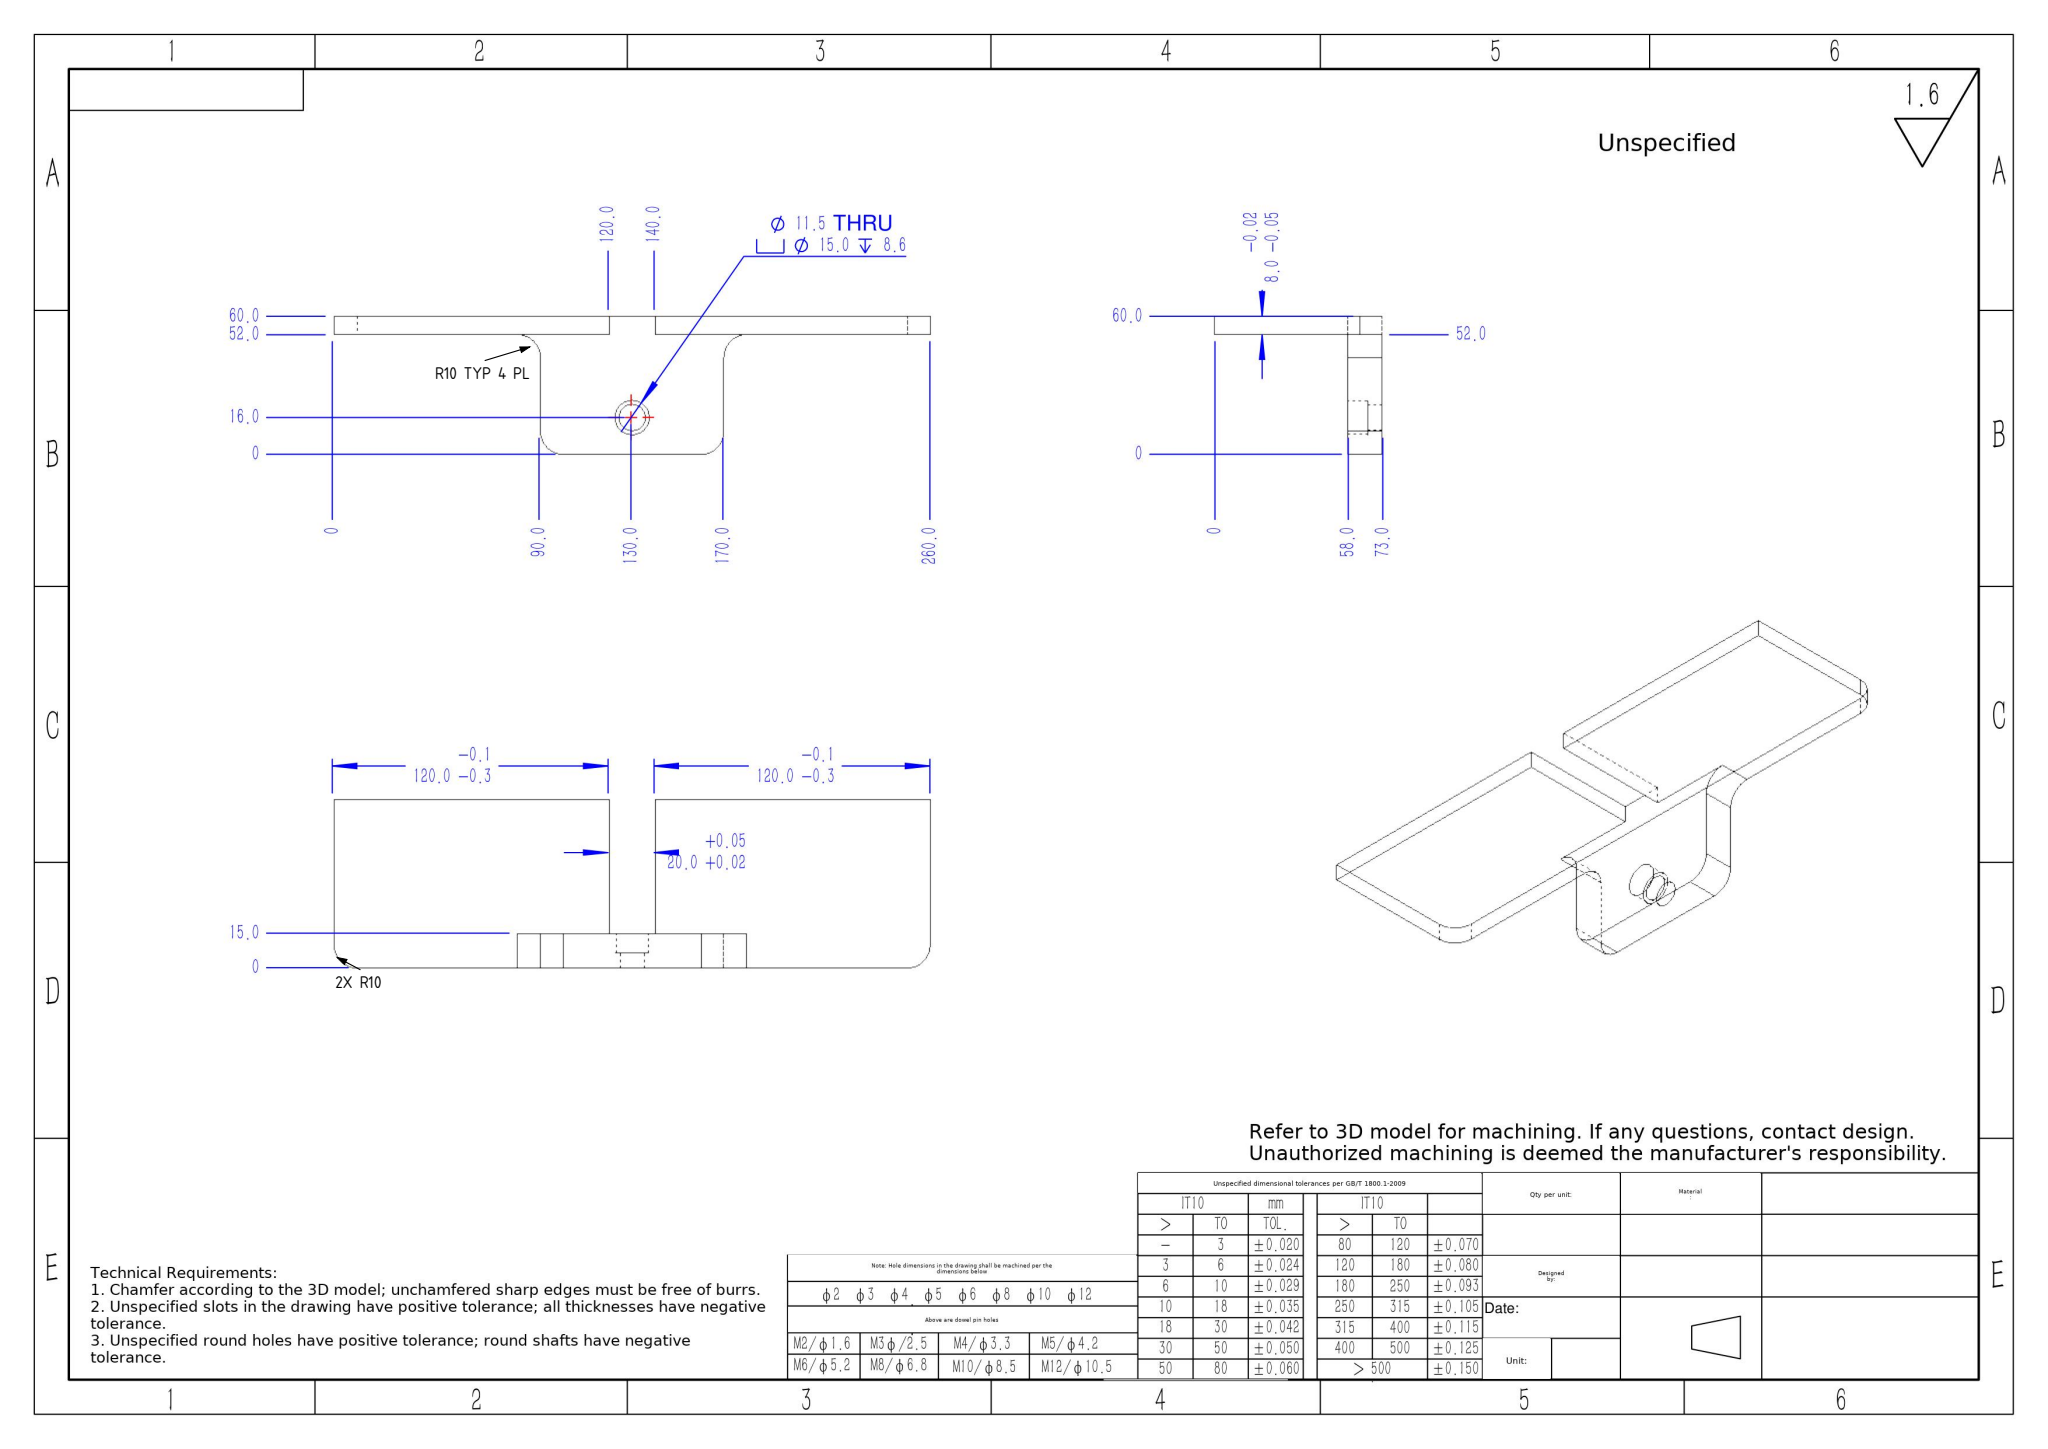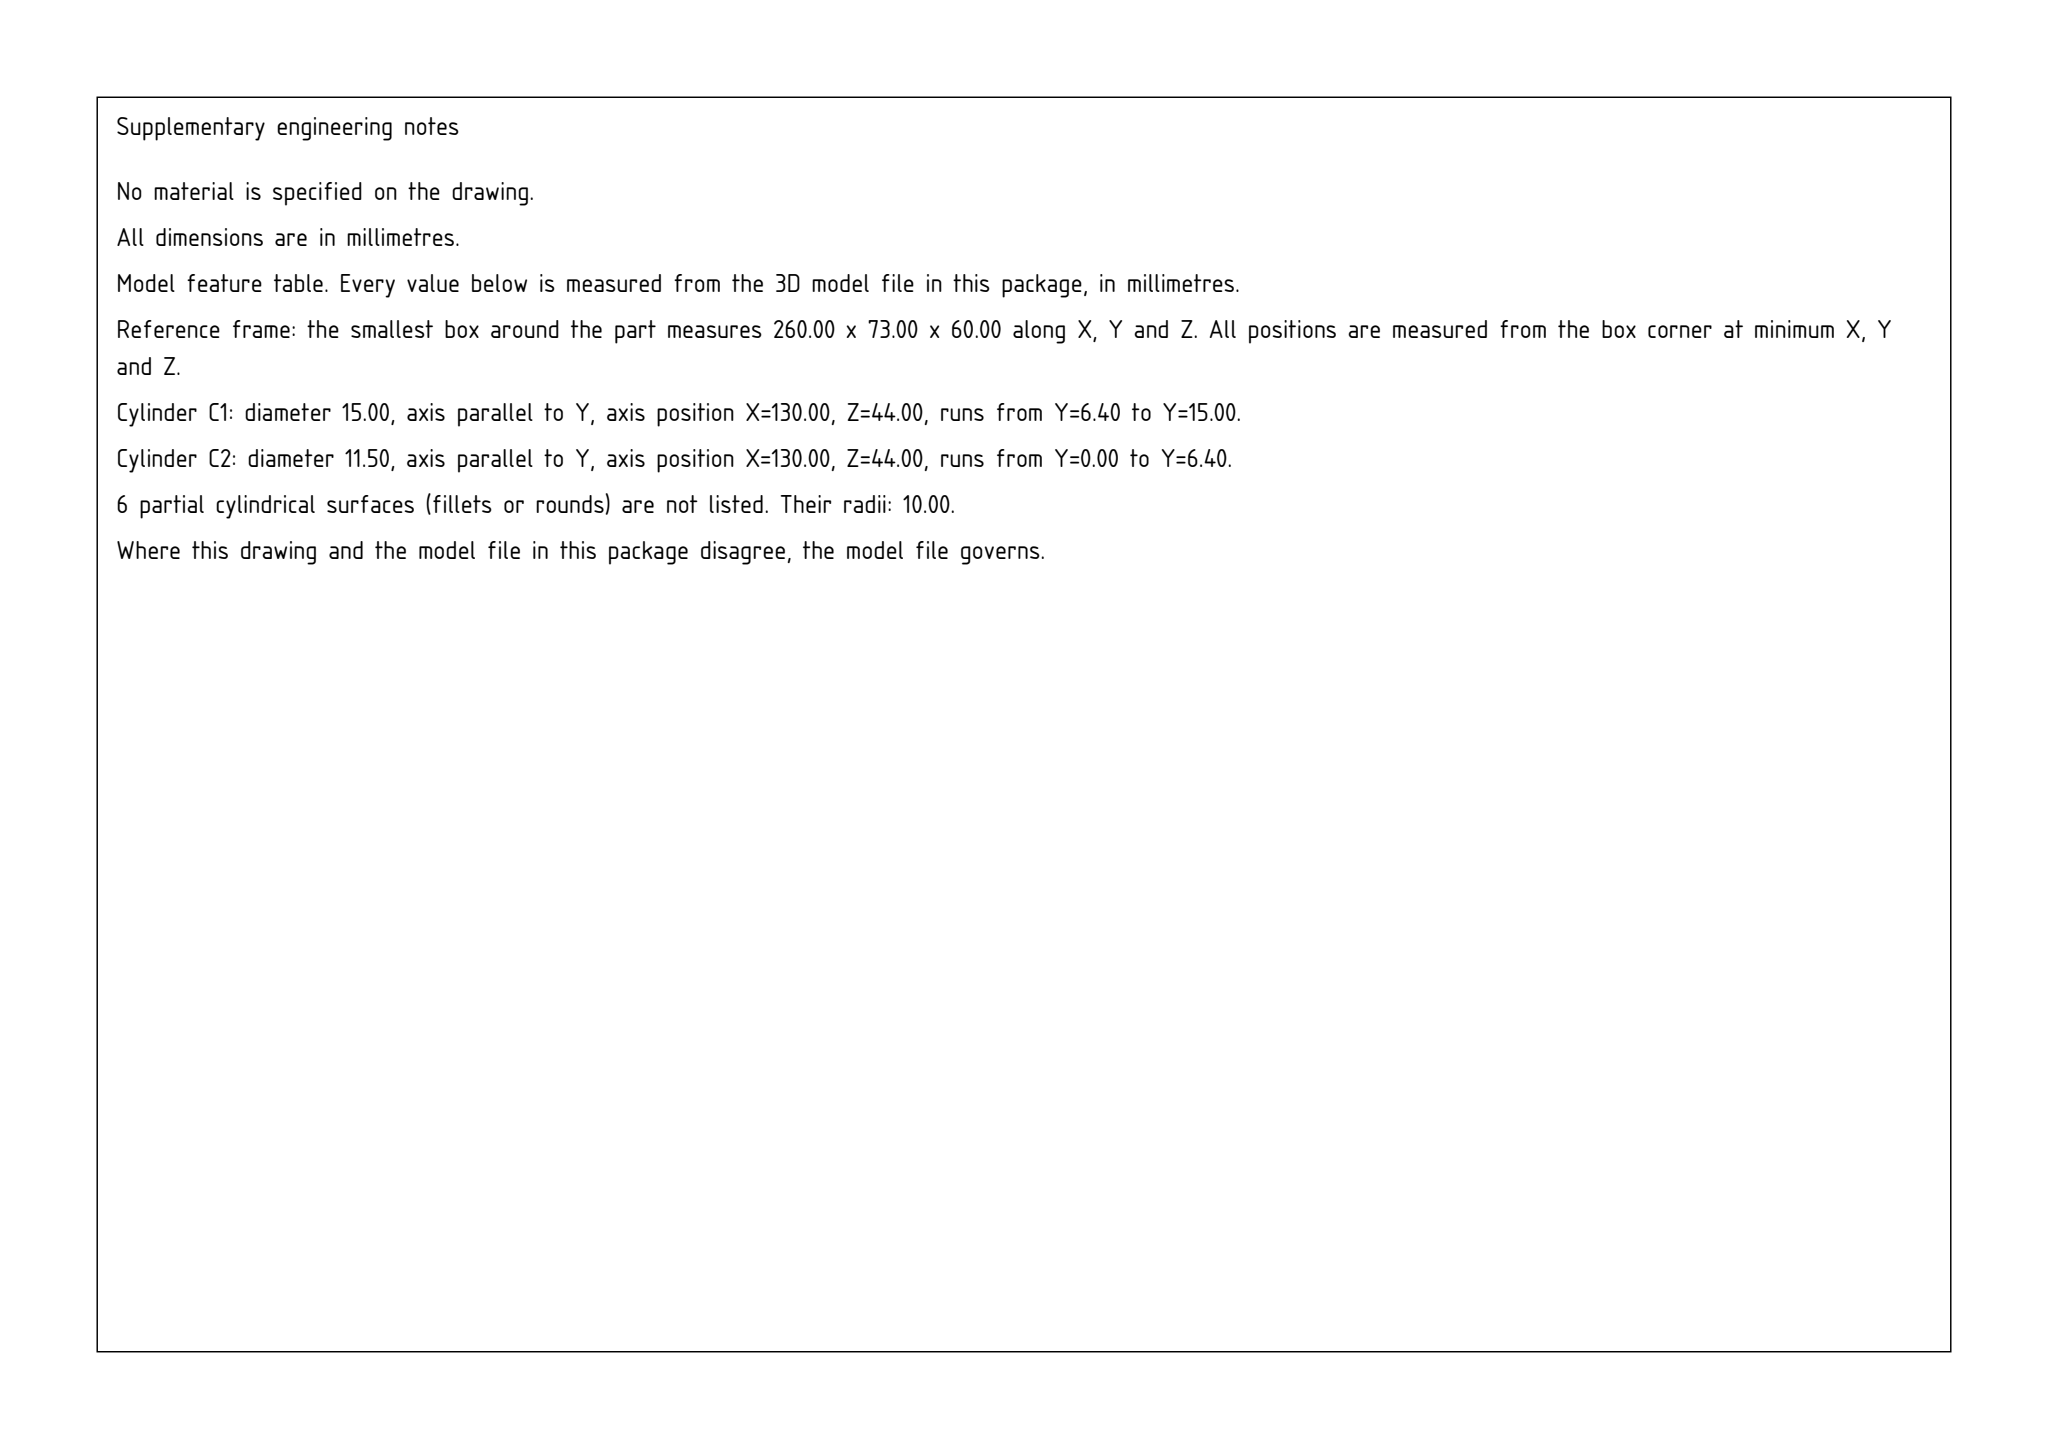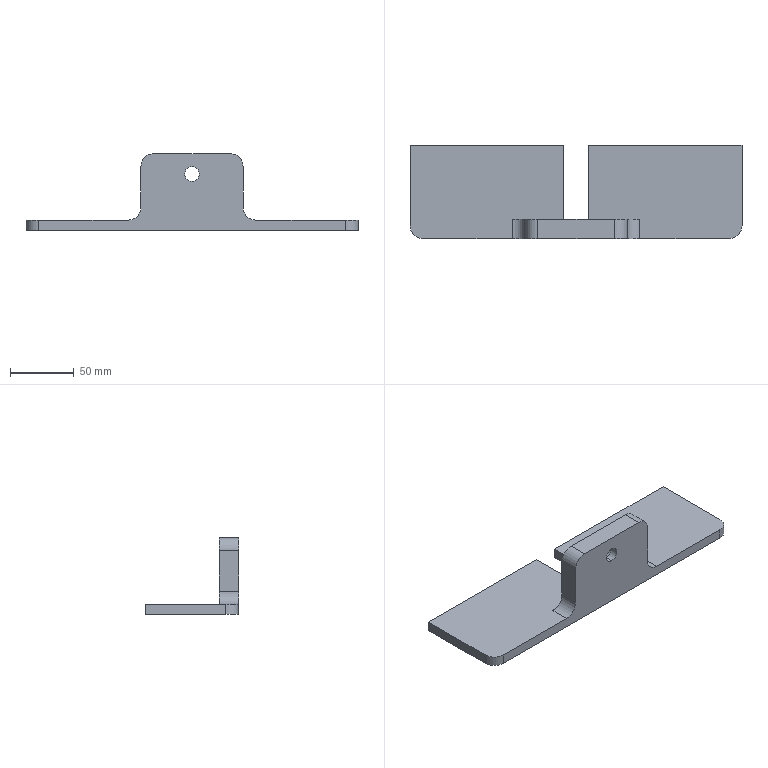Part | SolidWorks | mm | 1 solid | 25 faces | box 260 x 73 x 60 mm | volume 202432 mm3 | plane 15 | cylinder 10 | commonest cylinder face diameters 20 x6 15 x2 11.5 x2
Drawing notes:
R10 TYP 4 PL: WEB-TO-8 THK STRIP BLEND AT X=90 & X=170 | from the solid: cylinders dia 20, axis y, at (x,z)=(80,18),(100,50),(160,50),(180,18), len 15 -> R10 tangent to z=8/z=60 and x=90/170
FRONT VIEW: R10 AT 2 OUTER CORNERS OF 8 THK PLATE (X=0 & 260) | from the solid: cylinders dia 20, axis z, at (x,y)=(10,10),(250,10), len 8 -> R10 tangent to x=0/260 and y=0, thru 8 thk plate
build123d program:
from build123d import *

# Parameters (mm, degrees)
SKETCH1_W                                       = 260
SKETCH1_H                                       = 73
BOSS_EXTRUDE1_DEPTH                             = 30
SKETCH2_W                                       = 52
SKETCH2_H                                       = 58
CUT_EXTRUDE1_DEPTH                              = 265.258
SKETCH3_W                                       = 20
SKETCH3_H                                       = 58
CUT_EXTRUDE2_DEPTH                              = 10
SKETCH4_W                                       = 90
SKETCH4_H                                       = 52
CUT_EXTRUDE3_DEPTH                              = 32
FILLET1_R                                       = 10
FILLET2_R                                       = 10
M8_HEX_SOCKET_HEAD_CAP_SCREW_CBORE1_D           = 11.5
M8_HEX_SOCKET_HEAD_CAP_SCREW_CBORE1_CBORE_D     = 15
M8_HEX_SOCKET_HEAD_CAP_SCREW_CBORE1_CBORE_DEPTH = 8.6


with BuildPart() as part:
    # Sketch1 → Boss-Extrude1 (new, symmetric)
    with BuildSketch(Plane.XY):
        Rectangle(SKETCH1_W, SKETCH1_H)
    extrude(amount=BOSS_EXTRUDE1_DEPTH, both=True)

    # Sketch2 → Cut-Extrude1 (cut, through all)
    with BuildSketch(Plane.ZY.offset(130)):
        with Locations((4, 7.5)):
            Rectangle(SKETCH2_W, SKETCH2_H)
    extrude(amount=-CUT_EXTRUDE1_DEPTH, mode=Mode.SUBTRACT)

    # Sketch3 → Cut-Extrude2 (cut)
    with BuildSketch(Plane.XY.offset(-22)):
        with Locations((0, 7.5)):
            Rectangle(SKETCH3_W, SKETCH3_H)
    extrude(amount=-CUT_EXTRUDE2_DEPTH, mode=Mode.SUBTRACT)

    # Sketch4 → Cut-Extrude3 (cut)
    with BuildSketch(Plane(origin=(0, -21.5, 0), x_dir=(1, 0, 0), z_dir=(0, 1, 0))):
        with Locations((85, -4)):
            Rectangle(SKETCH4_W, SKETCH4_H)
    cut_extrude3 = extrude(amount=-CUT_EXTRUDE3_DEPTH, mode=Mode.SUBTRACT)

    # Mirror1: Cut-Extrude3 across plane
    add(cut_extrude3.mirror(Plane(origin=(0, 0, 0), x_dir=(0, 0, 1), z_dir=(1, 0, 0))), mode=Mode.SUBTRACT)

    # Fillet1
    fillet1_edges = [part.edges().sort_by_distance(p)[0] for p in [
        (40, -29, -22),
        (-40, -29, -22),
    ]]
    fillet(fillet1_edges, radius=FILLET1_R)

    # Fillet2
    fillet2_edges = [part.edges().sort_by_distance(p)[0] for p in [
        (130, -36.5, -26),
        (40, -29, 30),
        (-130, -36.5, -26),
        (-40, -29, 30),
    ]]
    fillet(fillet2_edges, radius=FILLET2_R)

    # M8 Hex Socket Head Cap Screw CBORE1 (through all)
    with Locations(Plane(origin=(0, -21.5, 0), x_dir=(1, 0, 0), z_dir=(0, 1, 0))):
        with Locations((0, -14)):
            CounterBoreHole(M8_HEX_SOCKET_HEAD_CAP_SCREW_CBORE1_D / 2, M8_HEX_SOCKET_HEAD_CAP_SCREW_CBORE1_CBORE_D / 2, M8_HEX_SOCKET_HEAD_CAP_SCREW_CBORE1_CBORE_DEPTH)


solid = part.part
STEP:
#1=CARTESIAN_POINT('',(0.,-30.1,6.5));
#2=VERTEX_POINT('',#1);
#3=CARTESIAN_POINT('',(0.,-30.1,21.5));
#4=VERTEX_POINT('',#3);
#5=CARTESIAN_POINT('',(0.,-30.1,14.));
#6=DIRECTION('',(0.,1.,-0.));
#7=DIRECTION('',(0.,0.,1.));
#8=AXIS2_PLACEMENT_3D('',#5,#6,#7);
#9=CIRCLE('',#8,7.5);
#10=EDGE_CURVE('',#2,#4,#9,.T.);
#11=ORIENTED_EDGE('',*,*,#10,.F.);
#12=CARTESIAN_POINT('',(0.,-21.5,6.5));
#13=VERTEX_POINT('',#12);
#14=CARTESIAN_POINT('',(0.,-21.5,6.5));
#15=DIRECTION('',(0.,1.,-0.));
#16=VECTOR('',#15,1000.);
#17=LINE('',#14,#16);
#18=EDGE_CURVE('',#2,#13,#17,.T.);
#19=ORIENTED_EDGE('',*,*,#18,.T.);
#20=CARTESIAN_POINT('',(0.,-21.5,21.5));
#21=VERTEX_POINT('',#20);
#22=CARTESIAN_POINT('',(0.,-21.5,14.));
#23=DIRECTION('',(0.,1.,-0.));
#24=DIRECTION('',(0.,0.,1.));
#25=AXIS2_PLACEMENT_3D('',#22,#23,#24);
#26=CIRCLE('',#25,7.5);
#27=EDGE_CURVE('',#13,#21,#26,.T.);
#28=ORIENTED_EDGE('',*,*,#27,.T.);
#29=CARTESIAN_POINT('',(0.,-21.5,21.5));
#30=DIRECTION('',(0.,1.,-0.));
#31=VECTOR('',#30,1000.);
#32=LINE('',#29,#31);
#33=EDGE_CURVE('',#4,#21,#32,.T.);
#34=ORIENTED_EDGE('',*,*,#33,.F.);
#35=EDGE_LOOP('',(#11,#19,#28,#34));
#36=FACE_OUTER_BOUND('',#35,.T.);
#37=CARTESIAN_POINT('',(0.,-21.5,14.));
#38=DIRECTION('',(0.,1.,-0.));
#39=DIRECTION('',(0.,0.,1.));
#40=AXIS2_PLACEMENT_3D('',#37,#38,#39);
#41=CYLINDRICAL_SURFACE('',#40,7.5);
#42=ADVANCED_FACE('',(#36),#41,.F.);
#43=CARTESIAN_POINT('',(0.,-36.5,8.25));
#44=VERTEX_POINT('',#43);
#45=CARTESIAN_POINT('',(0.,-36.5,19.75));
#46=VERTEX_POINT('',#45);
#47=CARTESIAN_POINT('',(0.,-36.5,14.));
#48=DIRECTION('',(0.,1.,-0.));
#49=DIRECTION('',(0.,0.,1.));
#50=AXIS2_PLACEMENT_3D('',#47,#48,#49);
#51=CIRCLE('',#50,5.75);
#52=EDGE_CURVE('',#44,#46,#51,.T.);
#53=ORIENTED_EDGE('',*,*,#52,.F.);
#54=CARTESIAN_POINT('',(0.,-30.1,8.25));
#55=VERTEX_POINT('',#54);
#56=CARTESIAN_POINT('',(0.,-21.5,8.25));
#57=DIRECTION('',(0.,1.,-0.));
#58=VECTOR('',#57,1000.);
#59=LINE('',#56,#58);
#60=EDGE_CURVE('',#44,#55,#59,.T.);
#61=ORIENTED_EDGE('',*,*,#60,.T.);
#62=CARTESIAN_POINT('',(0.,-30.1,19.75));
#63=VERTEX_POINT('',#62);
#64=CARTESIAN_POINT('',(0.,-30.1,14.));
#65=DIRECTION('',(0.,1.,-0.));
#66=DIRECTION('',(0.,0.,1.));
#67=AXIS2_PLACEMENT_3D('',#64,#65,#66);
#68=CIRCLE('',#67,5.75);
#69=EDGE_CURVE('',#55,#63,#68,.T.);
#70=ORIENTED_EDGE('',*,*,#69,.T.);
#71=CARTESIAN_POINT('',(0.,-21.5,19.75));
#72=DIRECTION('',(0.,1.,-0.));
#73=VECTOR('',#72,1000.);
#74=LINE('',#71,#73);
#75=EDGE_CURVE('',#46,#63,#74,.T.);
#76=ORIENTED_EDGE('',*,*,#75,.F.);
#77=EDGE_LOOP('',(#53,#61,#70,#76));
#78=FACE_OUTER_BOUND('',#77,.T.);
#79=CARTESIAN_POINT('',(0.,-21.5,14.));
#80=DIRECTION('',(0.,1.,-0.));
#81=DIRECTION('',(0.,0.,1.));
#82=AXIS2_PLACEMENT_3D('',#79,#80,#81);
#83=CYLINDRICAL_SURFACE('',#82,5.75);
#84=ADVANCED_FACE('',(#78),#83,.F.);
#85=CARTESIAN_POINT('',(-130.,36.5,-30.));
#86=VERTEX_POINT('',#85);
#87=CARTESIAN_POINT('',(-130.,-26.5,-30.));
#88=VERTEX_POINT('',#87);
#89=CARTESIAN_POINT('',(-130.,-36.5,-30.));
#90=DIRECTION('',(0.,-1.,0.));
#91=VECTOR('',#90,1000.);
#92=LINE('',#89,#91);
#93=EDGE_CURVE('',#86,#88,#92,.T.);
#94=ORIENTED_EDGE('',*,*,#93,.T.);
#95=CARTESIAN_POINT('',(-130.,-26.5,-22.));
#96=VERTEX_POINT('',#95);
#97=CARTESIAN_POINT('',(-130.,-26.5,30.));
#98=DIRECTION('',(0.,0.,1.));
#99=VECTOR('',#98,1000.);
#100=LINE('',#97,#99);
#101=EDGE_CURVE('',#88,#96,#100,.T.);
#102=ORIENTED_EDGE('',*,*,#101,.T.);
#103=CARTESIAN_POINT('',(-130.,36.5,-22.));
#104=VERTEX_POINT('',#103);
#105=CARTESIAN_POINT('',(-130.,36.5,-22.));
#106=DIRECTION('',(0.,-1.,0.));
#107=VECTOR('',#106,1000.);
#108=LINE('',#105,#107);
#109=EDGE_CURVE('',#104,#96,#108,.T.);
#110=ORIENTED_EDGE('',*,*,#109,.F.);
#111=CARTESIAN_POINT('',(-130.,36.5,30.));
#112=DIRECTION('',(0.,0.,-1.));
#113=VECTOR('',#112,1000.);
#114=LINE('',#111,#113);
#115=EDGE_CURVE('',#104,#86,#114,.T.);
#116=ORIENTED_EDGE('',*,*,#115,.T.);
#117=EDGE_LOOP('',(#94,#102,#110,#116));
#118=FACE_OUTER_BOUND('',#117,.T.);
#119=CARTESIAN_POINT('',(-130.,-36.5,30.));
#120=DIRECTION('',(1.,0.,0.));
#121=DIRECTION('',(0.,0.,-1.));
#122=AXIS2_PLACEMENT_3D('',#119,#120,#121);
#123=PLANE('',#122);
#124=ADVANCED_FACE('',(#118),#123,.F.);
#125=CARTESIAN_POINT('',(0.,-36.5,14.));
#126=DIRECTION('',(0.,1.,-0.));
#127=DIRECTION('',(0.,0.,1.));
#128=AXIS2_PLACEMENT_3D('',#125,#126,#127);
#129=CIRCLE('',#128,5.75);
#130=EDGE_CURVE('',#46,#44,#129,.T.);
#131=ORIENTED_EDGE('',*,*,#130,.T.);
#132=ORIENTED_EDGE('',*,*,#52,.T.);
#133=EDGE_LOOP('',(#131,#132));
#134=FACE_BOUND('',#133,.T.);
#135=CARTESIAN_POINT('',(-30.,-36.5,30.));
#136=VERTEX_POINT('',#135);
#137=CARTESIAN_POINT('',(30.,-36.5,30.));
#138=VERTEX_POINT('',#137);
#139=CARTESIAN_POINT('',(-130.,-36.5,30.));
#140=DIRECTION('',(1.,0.,0.));
#141=VECTOR('',#140,1000.);
#142=LINE('',#139,#141);
#143=EDGE_CURVE('',#136,#138,#142,.T.);
#144=ORIENTED_EDGE('',*,*,#143,.F.);
#145=CARTESIAN_POINT('',(-40.,-36.5,20.));
#146=VERTEX_POINT('',#145);
#147=CARTESIAN_POINT('',(-30.,-36.5,20.));
#148=DIRECTION('',(0.,-1.,0.));
#149=DIRECTION('',(0.,0.,1.));
#150=AXIS2_PLACEMENT_3D('',#147,#148,#149);
#151=CIRCLE('',#150,10.);
#152=EDGE_CURVE('',#136,#146,#151,.T.);
#153=ORIENTED_EDGE('',*,*,#152,.T.);
#154=CARTESIAN_POINT('',(-40.,-36.5,-12.));
#155=VERTEX_POINT('',#154);
#156=CARTESIAN_POINT('',(-40.,-36.5,30.));
#157=DIRECTION('',(0.,0.,1.));
#158=VECTOR('',#157,1000.);
#159=LINE('',#156,#158);
#160=EDGE_CURVE('',#155,#146,#159,.T.);
#161=ORIENTED_EDGE('',*,*,#160,.F.);
#162=CARTESIAN_POINT('',(-50.,-36.5,-22.));
#163=VERTEX_POINT('',#162);
#164=CARTESIAN_POINT('',(-50.,-36.5,-12.));
#165=DIRECTION('',(0.,1.,0.));
#166=DIRECTION('',(0.,0.,1.));
#167=AXIS2_PLACEMENT_3D('',#164,#165,#166);
#168=CIRCLE('',#167,10.);
#169=EDGE_CURVE('',#155,#163,#168,.T.);
#170=ORIENTED_EDGE('',*,*,#169,.T.);
#171=CARTESIAN_POINT('',(-120.,-36.5,-22.));
#172=VERTEX_POINT('',#171);
#173=CARTESIAN_POINT('',(-130.,-36.5,-22.));
#174=DIRECTION('',(1.,0.,0.));
#175=VECTOR('',#174,1000.);
#176=LINE('',#173,#175);
#177=EDGE_CURVE('',#172,#163,#176,.T.);
#178=ORIENTED_EDGE('',*,*,#177,.F.);
#179=CARTESIAN_POINT('',(-120.,-36.5,-30.));
#180=VERTEX_POINT('',#179);
#181=CARTESIAN_POINT('',(-120.,-36.5,30.));
#182=DIRECTION('',(0.,0.,-1.));
#183=VECTOR('',#182,1000.);
#184=LINE('',#181,#183);
#185=EDGE_CURVE('',#172,#180,#184,.T.);
#186=ORIENTED_EDGE('',*,*,#185,.T.);
#187=CARTESIAN_POINT('',(120.,-36.5,-30.));
#188=VERTEX_POINT('',#187);
#189=CARTESIAN_POINT('',(-130.,-36.5,-30.));
#190=DIRECTION('',(1.,0.,0.));
#191=VECTOR('',#190,1000.);
#192=LINE('',#189,#191);
#193=EDGE_CURVE('',#180,#188,#192,.T.);
#194=ORIENTED_EDGE('',*,*,#193,.T.);
#195=CARTESIAN_POINT('',(120.,-36.5,-22.));
#196=VERTEX_POINT('',#195);
#197=CARTESIAN_POINT('',(120.,-36.5,30.));
#198=DIRECTION('',(0.,0.,1.));
#199=VECTOR('',#198,1000.);
#200=LINE('',#197,#199);
#201=EDGE_CURVE('',#188,#196,#200,.T.);
#202=ORIENTED_EDGE('',*,*,#201,.T.);
#203=CARTESIAN_POINT('',(50.,-36.5,-22.));
#204=VERTEX_POINT('',#203);
#205=CARTESIAN_POINT('',(-130.,-36.5,-22.));
#206=DIRECTION('',(-1.,0.,0.));
#207=VECTOR('',#206,1000.);
#208=LINE('',#205,#207);
#209=EDGE_CURVE('',#196,#204,#208,.T.);
#210=ORIENTED_EDGE('',*,*,#209,.T.);
#211=CARTESIAN_POINT('',(40.,-36.5,-12.));
#212=VERTEX_POINT('',#211);
#213=CARTESIAN_POINT('',(50.,-36.5,-12.));
#214=DIRECTION('',(0.,1.,0.));
#215=DIRECTION('',(0.,0.,1.));
#216=AXIS2_PLACEMENT_3D('',#213,#214,#215);
#217=CIRCLE('',#216,10.);
#218=EDGE_CURVE('',#204,#212,#217,.T.);
#219=ORIENTED_EDGE('',*,*,#218,.T.);
#220=CARTESIAN_POINT('',(40.,-36.5,20.));
#221=VERTEX_POINT('',#220);
#222=CARTESIAN_POINT('',(40.,-36.5,30.));
#223=DIRECTION('',(0.,0.,1.));
#224=VECTOR('',#223,1000.);
#225=LINE('',#222,#224);
#226=EDGE_CURVE('',#212,#221,#225,.T.);
#227=ORIENTED_EDGE('',*,*,#226,.T.);
#228=CARTESIAN_POINT('',(30.,-36.5,20.));
#229=DIRECTION('',(0.,-1.,0.));
#230=DIRECTION('',(0.,0.,1.));
#231=AXIS2_PLACEMENT_3D('',#228,#229,#230);
#232=CIRCLE('',#231,10.);
#233=EDGE_CURVE('',#221,#138,#232,.T.);
#234=ORIENTED_EDGE('',*,*,#233,.T.);
#235=EDGE_LOOP('',(#144,#153,#161,#170,#178,#186,#194,#202,#210,#219,#227,#234));
#236=FACE_OUTER_BOUND('',#235,.T.);
#237=CARTESIAN_POINT('',(-130.,-36.5,30.));
#238=DIRECTION('',(0.,1.,0.));
#239=DIRECTION('',(0.,0.,1.));
#240=AXIS2_PLACEMENT_3D('',#237,#238,#239);
#241=PLANE('',#240);
#242=ADVANCED_FACE('',(#134,#236),#241,.F.);
#243=CARTESIAN_POINT('',(30.,-21.5,30.));
#244=VERTEX_POINT('',#243);
#245=CARTESIAN_POINT('',(-30.,-21.5,30.));
#246=VERTEX_POINT('',#245);
#247=CARTESIAN_POINT('',(130.,-21.5,30.));
#248=DIRECTION('',(-1.,0.,0.));
#249=VECTOR('',#248,1000.);
#250=LINE('',#247,#249);
#251=EDGE_CURVE('',#244,#246,#250,.T.);
#252=ORIENTED_EDGE('',*,*,#251,.T.);
#253=CARTESIAN_POINT('',(-30.,-36.5,30.));
#254=DIRECTION('',(0.,-1.,0.));
#255=VECTOR('',#254,1000.);
#256=LINE('',#253,#255);
#257=EDGE_CURVE('',#246,#136,#256,.T.);
#258=ORIENTED_EDGE('',*,*,#257,.T.);
#259=ORIENTED_EDGE('',*,*,#143,.T.);
#260=CARTESIAN_POINT('',(30.,0.,30.));
#261=DIRECTION('',(0.,1.,0.));
#262=VECTOR('',#261,1000.);
#263=LINE('',#260,#262);
#264=EDGE_CURVE('',#138,#244,#263,.T.);
#265=ORIENTED_EDGE('',*,*,#264,.T.);
#266=EDGE_LOOP('',(#252,#258,#259,#265));
#267=FACE_OUTER_BOUND('',#266,.T.);
#268=CARTESIAN_POINT('',(0.,0.,30.));
#269=DIRECTION('',(0.,0.,-1.));
#270=DIRECTION('',(-1.,0.,0.));
#271=AXIS2_PLACEMENT_3D('',#268,#269,#270);
#272=PLANE('',#271);
#273=ADVANCED_FACE('',(#267),#272,.F.);
#274=CARTESIAN_POINT('',(0.,-21.5,14.));
#275=DIRECTION('',(0.,1.,-0.));
#276=DIRECTION('',(0.,0.,1.));
#277=AXIS2_PLACEMENT_3D('',#274,#275,#276);
#278=CIRCLE('',#277,7.5);
#279=EDGE_CURVE('',#21,#13,#278,.T.);
#280=ORIENTED_EDGE('',*,*,#279,.F.);
#281=ORIENTED_EDGE('',*,*,#27,.F.);
#282=EDGE_LOOP('',(#280,#281));
#283=FACE_BOUND('',#282,.T.);
#284=CARTESIAN_POINT('',(-40.,-21.5,-12.));
#285=VERTEX_POINT('',#284);
#286=CARTESIAN_POINT('',(-40.,-21.5,20.));
#287=VERTEX_POINT('',#286);
#288=CARTESIAN_POINT('',(-40.,-21.5,30.));
#289=DIRECTION('',(0.,0.,1.));
#290=VECTOR('',#289,1000.);
#291=LINE('',#288,#290);
#292=EDGE_CURVE('',#285,#287,#291,.T.);
#293=ORIENTED_EDGE('',*,*,#292,.T.);
#294=CARTESIAN_POINT('',(-30.,-21.5,20.));
#295=DIRECTION('',(0.,1.,-0.));
#296=DIRECTION('',(0.,0.,-1.));
#297=AXIS2_PLACEMENT_3D('',#294,#295,#296);
#298=CIRCLE('',#297,10.);
#299=EDGE_CURVE('',#287,#246,#298,.T.);
#300=ORIENTED_EDGE('',*,*,#299,.T.);
#301=ORIENTED_EDGE('',*,*,#251,.F.);
#302=CARTESIAN_POINT('',(40.,-21.5,20.));
#303=VERTEX_POINT('',#302);
#304=CARTESIAN_POINT('',(30.,-21.5,20.));
#305=DIRECTION('',(0.,1.,-0.));
#306=DIRECTION('',(0.,0.,-1.));
#307=AXIS2_PLACEMENT_3D('',#304,#305,#306);
#308=CIRCLE('',#307,10.);
#309=EDGE_CURVE('',#244,#303,#308,.T.);
#310=ORIENTED_EDGE('',*,*,#309,.T.);
#311=CARTESIAN_POINT('',(40.,-21.5,-12.));
#312=VERTEX_POINT('',#311);
#313=CARTESIAN_POINT('',(40.,-21.5,30.));
#314=DIRECTION('',(0.,0.,1.));
#315=VECTOR('',#314,1000.);
#316=LINE('',#313,#315);
#317=EDGE_CURVE('',#312,#303,#316,.T.);
#318=ORIENTED_EDGE('',*,*,#317,.F.);
#319=CARTESIAN_POINT('',(50.,-21.5,-22.));
#320=VERTEX_POINT('',#319);
#321=CARTESIAN_POINT('',(50.,-21.5,-12.));
#322=DIRECTION('',(0.,-1.,0.));
#323=DIRECTION('',(0.,0.,-1.));
#324=AXIS2_PLACEMENT_3D('',#321,#322,#323);
#325=CIRCLE('',#324,10.);
#326=EDGE_CURVE('',#312,#320,#325,.T.);
#327=ORIENTED_EDGE('',*,*,#326,.T.);
#328=CARTESIAN_POINT('',(10.,-21.5,-22.));
#329=VERTEX_POINT('',#328);
#330=CARTESIAN_POINT('',(130.,-21.5,-22.));
#331=DIRECTION('',(-1.,0.,0.));
#332=VECTOR('',#331,1000.);
#333=LINE('',#330,#332);
#334=EDGE_CURVE('',#320,#329,#333,.T.);
#335=ORIENTED_EDGE('',*,*,#334,.T.);
#336=CARTESIAN_POINT('',(10.,-21.5,-30.));
#337=VERTEX_POINT('',#336);
#338=CARTESIAN_POINT('',(10.,-21.5,-32.));
#339=DIRECTION('',(0.,0.,1.));
#340=VECTOR('',#339,1000.);
#341=LINE('',#338,#340);
#342=EDGE_CURVE('',#337,#329,#341,.T.);
#343=ORIENTED_EDGE('',*,*,#342,.F.);
#344=CARTESIAN_POINT('',(-10.,-21.5,-30.));
#345=VERTEX_POINT('',#344);
#346=CARTESIAN_POINT('',(0.,-21.5,-30.));
#347=DIRECTION('',(-1.,0.,0.));
#348=VECTOR('',#347,1000.);
#349=LINE('',#346,#348);
#350=EDGE_CURVE('',#337,#345,#349,.T.);
#351=ORIENTED_EDGE('',*,*,#350,.T.);
#352=CARTESIAN_POINT('',(-10.,-21.5,-22.));
#353=VERTEX_POINT('',#352);
#354=CARTESIAN_POINT('',(-10.,-21.5,-32.));
#355=DIRECTION('',(0.,0.,1.));
#356=VECTOR('',#355,1000.);
#357=LINE('',#354,#356);
#358=EDGE_CURVE('',#345,#353,#357,.T.);
#359=ORIENTED_EDGE('',*,*,#358,.T.);
#360=CARTESIAN_POINT('',(-50.,-21.5,-22.));
#361=VERTEX_POINT('',#360);
#362=CARTESIAN_POINT('',(130.,-21.5,-22.));
#363=DIRECTION('',(-1.,0.,0.));
#364=VECTOR('',#363,1000.);
#365=LINE('',#362,#364);
#366=EDGE_CURVE('',#353,#361,#365,.T.);
#367=ORIENTED_EDGE('',*,*,#366,.T.);
#368=CARTESIAN_POINT('',(-50.,-21.5,-12.));
#369=DIRECTION('',(0.,-1.,0.));
#370=DIRECTION('',(0.,0.,-1.));
#371=AXIS2_PLACEMENT_3D('',#368,#369,#370);
#372=CIRCLE('',#371,10.);
#373=EDGE_CURVE('',#361,#285,#372,.T.);
#374=ORIENTED_EDGE('',*,*,#373,.T.);
#375=EDGE_LOOP('',(#293,#300,#301,#310,#318,#327,#335,#343,#351,#359,#367,#374));
#376=FACE_OUTER_BOUND('',#375,.T.);
#377=CARTESIAN_POINT('',(130.,-21.5,30.));
#378=DIRECTION('',(0.,-1.,0.));
#379=DIRECTION('',(0.,-0.,-1.));
#380=AXIS2_PLACEMENT_3D('',#377,#378,#379);
#381=PLANE('',#380);
#382=ADVANCED_FACE('',(#283,#376),#381,.F.);
#383=CARTESIAN_POINT('',(-10.,36.5,-22.));
#384=VERTEX_POINT('',#383);
#385=CARTESIAN_POINT('',(130.,36.5,-22.));
#386=DIRECTION('',(-1.,0.,0.));
#387=VECTOR('',#386,1000.);
#388=LINE('',#385,#387);
#389=EDGE_CURVE('',#384,#104,#388,.T.);
#390=ORIENTED_EDGE('',*,*,#389,.F.);
#391=CARTESIAN_POINT('',(-10.,36.5,-30.));
#392=VERTEX_POINT('',#391);
#393=CARTESIAN_POINT('',(-10.,36.5,-32.));
#394=DIRECTION('',(0.,0.,1.));
#395=VECTOR('',#394,1000.);
#396=LINE('',#393,#395);
#397=EDGE_CURVE('',#392,#384,#396,.T.);
#398=ORIENTED_EDGE('',*,*,#397,.F.);
#399=CARTESIAN_POINT('',(-130.,36.5,-30.));
#400=DIRECTION('',(-1.,0.,0.));
#401=VECTOR('',#400,1000.);
#402=LINE('',#399,#401);
#403=EDGE_CURVE('',#392,#86,#402,.T.);
#404=ORIENTED_EDGE('',*,*,#403,.T.);
#405=ORIENTED_EDGE('',*,*,#115,.F.);
#406=EDGE_LOOP('',(#390,#398,#404,#405));
#407=FACE_OUTER_BOUND('',#406,.T.);
#408=CARTESIAN_POINT('',(-130.,36.5,30.));
#409=DIRECTION('',(0.,-1.,0.));
#410=DIRECTION('',(0.,0.,-1.));
#411=AXIS2_PLACEMENT_3D('',#408,#409,#410);
#412=PLANE('',#411);
#413=ADVANCED_FACE('',(#407),#412,.F.);
#414=ORIENTED_EDGE('',*,*,#109,.T.);
#415=CARTESIAN_POINT('',(-120.,-26.5,-22.));
#416=DIRECTION('',(0.,0.,1.));
#417=DIRECTION('',(0.,1.,0.));
#418=AXIS2_PLACEMENT_3D('',#415,#416,#417);
#419=CIRCLE('',#418,10.);
#420=EDGE_CURVE('',#96,#172,#419,.T.);
#421=ORIENTED_EDGE('',*,*,#420,.T.);
#422=ORIENTED_EDGE('',*,*,#177,.T.);
#423=CARTESIAN_POINT('',(-50.,36.5,-22.));
#424=DIRECTION('',(0.,1.,-0.));
#425=VECTOR('',#424,1000.);
#426=LINE('',#423,#425);
#427=EDGE_CURVE('',#163,#361,#426,.T.);
#428=ORIENTED_EDGE('',*,*,#427,.T.);
#429=ORIENTED_EDGE('',*,*,#366,.F.);
#430=CARTESIAN_POINT('',(-10.,36.5,-22.));
#431=DIRECTION('',(0.,-1.,0.));
#432=VECTOR('',#431,1000.);
#433=LINE('',#430,#432);
#434=EDGE_CURVE('',#384,#353,#433,.T.);
#435=ORIENTED_EDGE('',*,*,#434,.F.);
#436=ORIENTED_EDGE('',*,*,#389,.T.);
#437=EDGE_LOOP('',(#414,#421,#422,#428,#429,#435,#436));
#438=FACE_OUTER_BOUND('',#437,.T.);
#439=CARTESIAN_POINT('',(130.,36.5,-22.));
#440=DIRECTION('',(0.,-0.,-1.));
#441=DIRECTION('',(0.,1.,-0.));
#442=AXIS2_PLACEMENT_3D('',#439,#440,#441);
#443=PLANE('',#442);
#444=ADVANCED_FACE('',(#438),#443,.F.);
#445=CARTESIAN_POINT('',(130.,36.5,-22.));
#446=VERTEX_POINT('',#445);
#447=CARTESIAN_POINT('',(130.,-26.5,-22.));
#448=VERTEX_POINT('',#447);
#449=CARTESIAN_POINT('',(130.,36.5,-22.));
#450=DIRECTION('',(0.,-1.,0.));
#451=VECTOR('',#450,1000.);
#452=LINE('',#449,#451);
#453=EDGE_CURVE('',#446,#448,#452,.T.);
#454=ORIENTED_EDGE('',*,*,#453,.T.);
#455=CARTESIAN_POINT('',(130.,-26.5,-30.));
#456=VERTEX_POINT('',#455);
#457=CARTESIAN_POINT('',(130.,-26.5,30.));
#458=DIRECTION('',(0.,0.,-1.));
#459=VECTOR('',#458,1000.);
#460=LINE('',#457,#459);
#461=EDGE_CURVE('',#448,#456,#460,.T.);
#462=ORIENTED_EDGE('',*,*,#461,.T.);
#463=CARTESIAN_POINT('',(130.,36.5,-30.));
#464=VERTEX_POINT('',#463);
#465=CARTESIAN_POINT('',(130.,-36.5,-30.));
#466=DIRECTION('',(0.,1.,0.));
#467=VECTOR('',#466,1000.);
#468=LINE('',#465,#467);
#469=EDGE_CURVE('',#456,#464,#468,.T.);
#470=ORIENTED_EDGE('',*,*,#469,.T.);
#471=CARTESIAN_POINT('',(130.,36.5,30.));
#472=DIRECTION('',(0.,0.,-1.));
#473=VECTOR('',#472,1000.);
#474=LINE('',#471,#473);
#475=EDGE_CURVE('',#446,#464,#474,.T.);
#476=ORIENTED_EDGE('',*,*,#475,.F.);
#477=EDGE_LOOP('',(#454,#462,#470,#476));
#478=FACE_OUTER_BOUND('',#477,.T.);
#479=CARTESIAN_POINT('',(130.,-36.5,30.));
#480=DIRECTION('',(-1.,0.,0.));
#481=DIRECTION('',(0.,0.,1.));
#482=AXIS2_PLACEMENT_3D('',#479,#480,#481);
#483=PLANE('',#482);
#484=ADVANCED_FACE('',(#478),#483,.F.);
#485=CARTESIAN_POINT('',(10.,36.5,-30.));
#486=VERTEX_POINT('',#485);
#487=CARTESIAN_POINT('',(-130.,36.5,-30.));
#488=DIRECTION('',(-1.,0.,0.));
#489=VECTOR('',#488,1000.);
#490=LINE('',#487,#489);
#491=EDGE_CURVE('',#464,#486,#490,.T.);
#492=ORIENTED_EDGE('',*,*,#491,.T.);
#493=CARTESIAN_POINT('',(10.,36.5,-22.));
#494=VERTEX_POINT('',#493);
#495=CARTESIAN_POINT('',(10.,36.5,-32.));
#496=DIRECTION('',(0.,0.,1.));
#497=VECTOR('',#496,1000.);
#498=LINE('',#495,#497);
#499=EDGE_CURVE('',#486,#494,#498,.T.);
#500=ORIENTED_EDGE('',*,*,#499,.T.);
#501=CARTESIAN_POINT('',(130.,36.5,-22.));
#502=DIRECTION('',(-1.,0.,0.));
#503=VECTOR('',#502,1000.);
#504=LINE('',#501,#503);
#505=EDGE_CURVE('',#446,#494,#504,.T.);
#506=ORIENTED_EDGE('',*,*,#505,.F.);
#507=ORIENTED_EDGE('',*,*,#475,.T.);
#508=EDGE_LOOP('',(#492,#500,#506,#507));
#509=FACE_OUTER_BOUND('',#508,.T.);
#510=CARTESIAN_POINT('',(-130.,36.5,30.));
#511=DIRECTION('',(0.,-1.,0.));
#512=DIRECTION('',(0.,0.,-1.));
#513=AXIS2_PLACEMENT_3D('',#510,#511,#512);
#514=PLANE('',#513);
#515=ADVANCED_FACE('',(#509),#514,.F.);
#516=ORIENTED_EDGE('',*,*,#193,.F.);
#517=CARTESIAN_POINT('',(-120.,-26.5,-30.));
#518=DIRECTION('',(0.,0.,-1.));
#519=DIRECTION('',(-1.,0.,0.));
#520=AXIS2_PLACEMENT_3D('',#517,#518,#519);
#521=CIRCLE('',#520,10.);
#522=EDGE_CURVE('',#180,#88,#521,.T.);
#523=ORIENTED_EDGE('',*,*,#522,.T.);
#524=ORIENTED_EDGE('',*,*,#93,.F.);
#525=ORIENTED_EDGE('',*,*,#403,.F.);
#526=CARTESIAN_POINT('',(-10.,-0.,-30.));
#527=DIRECTION('',(-0.,1.,0.));
#528=VECTOR('',#527,1000.);
#529=LINE('',#526,#528);
#530=EDGE_CURVE('',#345,#392,#529,.T.);
#531=ORIENTED_EDGE('',*,*,#530,.F.);
#532=ORIENTED_EDGE('',*,*,#350,.F.);
#533=CARTESIAN_POINT('',(10.,-0.,-30.));
#534=DIRECTION('',(-0.,-1.,0.));
#535=VECTOR('',#534,1000.);
#536=LINE('',#533,#535);
#537=EDGE_CURVE('',#486,#337,#536,.T.);
#538=ORIENTED_EDGE('',*,*,#537,.F.);
#539=ORIENTED_EDGE('',*,*,#491,.F.);
#540=ORIENTED_EDGE('',*,*,#469,.F.);
#541=CARTESIAN_POINT('',(120.,-26.5,-30.));
#542=DIRECTION('',(0.,0.,-1.));
#543=DIRECTION('',(-1.,0.,0.));
#544=AXIS2_PLACEMENT_3D('',#541,#542,#543);
#545=CIRCLE('',#544,10.);
#546=EDGE_CURVE('',#456,#188,#545,.T.);
#547=ORIENTED_EDGE('',*,*,#546,.T.);
#548=EDGE_LOOP('',(#516,#523,#524,#525,#531,#532,#538,#539,#540,#547));
#549=FACE_OUTER_BOUND('',#548,.T.);
#550=CARTESIAN_POINT('',(0.,0.,-30.));
#551=DIRECTION('',(0.,0.,-1.));
#552=DIRECTION('',(-1.,0.,0.));
#553=AXIS2_PLACEMENT_3D('',#550,#551,#552);
#554=PLANE('',#553);
#555=ADVANCED_FACE('',(#549),#554,.T.);
#556=ORIENTED_EDGE('',*,*,#209,.F.);
#557=CARTESIAN_POINT('',(120.,-26.5,-22.));
#558=DIRECTION('',(0.,0.,1.));
#559=DIRECTION('',(0.,1.,0.));
#560=AXIS2_PLACEMENT_3D('',#557,#558,#559);
#561=CIRCLE('',#560,10.);
#562=EDGE_CURVE('',#196,#448,#561,.T.);
#563=ORIENTED_EDGE('',*,*,#562,.T.);
#564=ORIENTED_EDGE('',*,*,#453,.F.);
#565=ORIENTED_EDGE('',*,*,#505,.T.);
#566=CARTESIAN_POINT('',(10.,36.5,-22.));
#567=DIRECTION('',(0.,1.,0.));
#568=VECTOR('',#567,1000.);
#569=LINE('',#566,#568);
#570=EDGE_CURVE('',#329,#494,#569,.T.);
#571=ORIENTED_EDGE('',*,*,#570,.F.);
#572=ORIENTED_EDGE('',*,*,#334,.F.);
#573=CARTESIAN_POINT('',(50.,-36.5,-22.));
#574=DIRECTION('',(0.,-1.,0.));
#575=VECTOR('',#574,1000.);
#576=LINE('',#573,#575);
#577=EDGE_CURVE('',#320,#204,#576,.T.);
#578=ORIENTED_EDGE('',*,*,#577,.T.);
#579=EDGE_LOOP('',(#556,#563,#564,#565,#571,#572,#578));
#580=FACE_OUTER_BOUND('',#579,.T.);
#581=CARTESIAN_POINT('',(130.,36.5,-22.));
#582=DIRECTION('',(0.,-0.,-1.));
#583=DIRECTION('',(0.,1.,-0.));
#584=AXIS2_PLACEMENT_3D('',#581,#582,#583);
#585=PLANE('',#584);
#586=ADVANCED_FACE('',(#580),#585,.F.);
#587=ORIENTED_EDGE('',*,*,#530,.T.);
#588=ORIENTED_EDGE('',*,*,#397,.T.);
#589=ORIENTED_EDGE('',*,*,#434,.T.);
#590=ORIENTED_EDGE('',*,*,#358,.F.);
#591=EDGE_LOOP('',(#587,#588,#589,#590));
#592=FACE_OUTER_BOUND('',#591,.T.);
#593=CARTESIAN_POINT('',(-10.,36.5,-32.));
#594=DIRECTION('',(-1.,-0.,0.));
#595=DIRECTION('',(0.,-1.,0.));
#596=AXIS2_PLACEMENT_3D('',#593,#594,#595);
#597=PLANE('',#596);
#598=ADVANCED_FACE('',(#592),#597,.F.);
#599=ORIENTED_EDGE('',*,*,#537,.T.);
#600=ORIENTED_EDGE('',*,*,#342,.T.);
#601=ORIENTED_EDGE('',*,*,#570,.T.);
#602=ORIENTED_EDGE('',*,*,#499,.F.);
#603=EDGE_LOOP('',(#599,#600,#601,#602));
#604=FACE_OUTER_BOUND('',#603,.T.);
#605=CARTESIAN_POINT('',(10.,36.5,-32.));
#606=DIRECTION('',(1.,-0.,0.));
#607=DIRECTION('',(0.,1.,0.));
#608=AXIS2_PLACEMENT_3D('',#605,#606,#607);
#609=PLANE('',#608);
#610=ADVANCED_FACE('',(#604),#609,.F.);
#611=ORIENTED_EDGE('',*,*,#317,.T.);
#612=CARTESIAN_POINT('',(40.,-53.5,20.));
#613=DIRECTION('',(0.,-1.,0.));
#614=VECTOR('',#613,1000.);
#615=LINE('',#612,#614);
#616=EDGE_CURVE('',#303,#221,#615,.T.);
#617=ORIENTED_EDGE('',*,*,#616,.T.);
#618=ORIENTED_EDGE('',*,*,#226,.F.);
#619=CARTESIAN_POINT('',(40.,-21.5,-12.));
#620=DIRECTION('',(0.,1.,-0.));
#621=VECTOR('',#620,1000.);
#622=LINE('',#619,#621);
#623=EDGE_CURVE('',#212,#312,#622,.T.);
#624=ORIENTED_EDGE('',*,*,#623,.T.);
#625=EDGE_LOOP('',(#611,#617,#618,#624));
#626=FACE_OUTER_BOUND('',#625,.T.);
#627=CARTESIAN_POINT('',(40.,-53.5,30.));
#628=DIRECTION('',(-1.,0.,0.));
#629=DIRECTION('',(0.,0.,1.));
#630=AXIS2_PLACEMENT_3D('',#627,#628,#629);
#631=PLANE('',#630);
#632=ADVANCED_FACE('',(#626),#631,.F.);
#633=ORIENTED_EDGE('',*,*,#160,.T.);
#634=CARTESIAN_POINT('',(-40.,-21.5,20.));
#635=DIRECTION('',(0.,1.,0.));
#636=VECTOR('',#635,1000.);
#637=LINE('',#634,#636);
#638=EDGE_CURVE('',#146,#287,#637,.T.);
#639=ORIENTED_EDGE('',*,*,#638,.T.);
#640=ORIENTED_EDGE('',*,*,#292,.F.);
#641=CARTESIAN_POINT('',(-40.,-53.5,-12.));
#642=DIRECTION('',(0.,-1.,0.));
#643=VECTOR('',#642,1000.);
#644=LINE('',#641,#643);
#645=EDGE_CURVE('',#285,#155,#644,.T.);
#646=ORIENTED_EDGE('',*,*,#645,.T.);
#647=EDGE_LOOP('',(#633,#639,#640,#646));
#648=FACE_OUTER_BOUND('',#647,.T.);
#649=CARTESIAN_POINT('',(-40.,-53.5,30.));
#650=DIRECTION('',(-1.,0.,0.));
#651=DIRECTION('',(0.,0.,1.));
#652=AXIS2_PLACEMENT_3D('',#649,#650,#651);
#653=PLANE('',#652);
#654=ADVANCED_FACE('',(#648),#653,.T.);
#655=ORIENTED_EDGE('',*,*,#169,.F.);
#656=ORIENTED_EDGE('',*,*,#645,.F.);
#657=ORIENTED_EDGE('',*,*,#373,.F.);
#658=ORIENTED_EDGE('',*,*,#427,.F.);
#659=EDGE_LOOP('',(#655,#656,#657,#658));
#660=FACE_OUTER_BOUND('',#659,.T.);
#661=CARTESIAN_POINT('',(-50.,36.5,-12.));
#662=DIRECTION('',(0.,1.,-0.));
#663=DIRECTION('',(0.,0.,1.));
#664=AXIS2_PLACEMENT_3D('',#661,#662,#663);
#665=CYLINDRICAL_SURFACE('',#664,10.);
#666=ADVANCED_FACE('',(#660),#665,.F.);
#667=ORIENTED_EDGE('',*,*,#218,.F.);
#668=ORIENTED_EDGE('',*,*,#577,.F.);
#669=ORIENTED_EDGE('',*,*,#326,.F.);
#670=ORIENTED_EDGE('',*,*,#623,.F.);
#671=EDGE_LOOP('',(#667,#668,#669,#670));
#672=FACE_OUTER_BOUND('',#671,.T.);
#673=CARTESIAN_POINT('',(50.,-53.5,-12.));
#674=DIRECTION('',(0.,-1.,0.));
#675=DIRECTION('',(0.,0.,-1.));
#676=AXIS2_PLACEMENT_3D('',#673,#674,#675);
#677=CYLINDRICAL_SURFACE('',#676,10.);
#678=ADVANCED_FACE('',(#672),#677,.F.);
#679=ORIENTED_EDGE('',*,*,#152,.F.);
#680=ORIENTED_EDGE('',*,*,#257,.F.);
#681=ORIENTED_EDGE('',*,*,#299,.F.);
#682=ORIENTED_EDGE('',*,*,#638,.F.);
#683=EDGE_LOOP('',(#679,#680,#681,#682));
#684=FACE_OUTER_BOUND('',#683,.T.);
#685=CARTESIAN_POINT('',(-30.,-53.5,20.));
#686=DIRECTION('',(0.,-1.,0.));
#687=DIRECTION('',(0.,0.,-1.));
#688=AXIS2_PLACEMENT_3D('',#685,#686,#687);
#689=CYLINDRICAL_SURFACE('',#688,10.);
#690=ADVANCED_FACE('',(#684),#689,.T.);
#691=ORIENTED_EDGE('',*,*,#233,.F.);
#692=ORIENTED_EDGE('',*,*,#616,.F.);
#693=ORIENTED_EDGE('',*,*,#309,.F.);
#694=ORIENTED_EDGE('',*,*,#264,.F.);
#695=EDGE_LOOP('',(#691,#692,#693,#694));
#696=FACE_OUTER_BOUND('',#695,.T.);
#697=CARTESIAN_POINT('',(30.,0.,20.));
#698=DIRECTION('',(0.,1.,0.));
#699=DIRECTION('',(0.,0.,1.));
#700=AXIS2_PLACEMENT_3D('',#697,#698,#699);
#701=CYLINDRICAL_SURFACE('',#700,10.);
#702=ADVANCED_FACE('',(#696),#701,.T.);
#703=ORIENTED_EDGE('',*,*,#420,.F.);
#704=ORIENTED_EDGE('',*,*,#101,.F.);
#705=ORIENTED_EDGE('',*,*,#522,.F.);
#706=ORIENTED_EDGE('',*,*,#185,.F.);
#707=EDGE_LOOP('',(#703,#704,#705,#706));
#708=FACE_OUTER_BOUND('',#707,.T.);
#709=CARTESIAN_POINT('',(-120.,-26.5,30.));
#710=DIRECTION('',(0.,0.,-1.));
#711=DIRECTION('',(-1.,0.,0.));
#712=AXIS2_PLACEMENT_3D('',#709,#710,#711);
#713=CYLINDRICAL_SURFACE('',#712,10.);
#714=ADVANCED_FACE('',(#708),#713,.T.);
#715=ORIENTED_EDGE('',*,*,#562,.F.);
#716=ORIENTED_EDGE('',*,*,#201,.F.);
#717=ORIENTED_EDGE('',*,*,#546,.F.);
#718=ORIENTED_EDGE('',*,*,#461,.F.);
#719=EDGE_LOOP('',(#715,#716,#717,#718));
#720=FACE_OUTER_BOUND('',#719,.T.);
#721=CARTESIAN_POINT('',(120.,-26.5,30.));
#722=DIRECTION('',(0.,0.,-1.));
#723=DIRECTION('',(-1.,0.,0.));
#724=AXIS2_PLACEMENT_3D('',#721,#722,#723);
#725=CYLINDRICAL_SURFACE('',#724,10.);
#726=ADVANCED_FACE('',(#720),#725,.T.);
#727=ORIENTED_EDGE('',*,*,#60,.F.);
#728=ORIENTED_EDGE('',*,*,#130,.F.);
#729=ORIENTED_EDGE('',*,*,#75,.T.);
#730=CARTESIAN_POINT('',(0.,-30.1,14.));
#731=DIRECTION('',(0.,1.,-0.));
#732=DIRECTION('',(0.,0.,1.));
#733=AXIS2_PLACEMENT_3D('',#730,#731,#732);
#734=CIRCLE('',#733,5.75);
#735=EDGE_CURVE('',#63,#55,#734,.T.);
#736=ORIENTED_EDGE('',*,*,#735,.T.);
#737=EDGE_LOOP('',(#727,#728,#729,#736));
#738=FACE_OUTER_BOUND('',#737,.T.);
#739=CARTESIAN_POINT('',(0.,-21.5,14.));
#740=DIRECTION('',(0.,1.,-0.));
#741=DIRECTION('',(0.,0.,1.));
#742=AXIS2_PLACEMENT_3D('',#739,#740,#741);
#743=CYLINDRICAL_SURFACE('',#742,5.75);
#744=ADVANCED_FACE('',(#738),#743,.F.);
#745=ORIENTED_EDGE('',*,*,#735,.F.);
#746=ORIENTED_EDGE('',*,*,#69,.F.);
#747=EDGE_LOOP('',(#745,#746));
#748=FACE_BOUND('',#747,.T.);
#749=CARTESIAN_POINT('',(0.,-30.1,14.));
#750=DIRECTION('',(0.,1.,-0.));
#751=DIRECTION('',(0.,0.,1.));
#752=AXIS2_PLACEMENT_3D('',#749,#750,#751);
#753=CIRCLE('',#752,7.5);
#754=EDGE_CURVE('',#4,#2,#753,.T.);
#755=ORIENTED_EDGE('',*,*,#754,.T.);
#756=ORIENTED_EDGE('',*,*,#10,.T.);
#757=EDGE_LOOP('',(#755,#756));
#758=FACE_OUTER_BOUND('',#757,.T.);
#759=CARTESIAN_POINT('',(5.75,-30.1,14.));
#760=DIRECTION('',(0.,-1.,0.));
#761=DIRECTION('',(0.,-0.,-1.));
#762=AXIS2_PLACEMENT_3D('',#759,#760,#761);
#763=PLANE('',#762);
#764=ADVANCED_FACE('',(#748,#758),#763,.F.);
#765=ORIENTED_EDGE('',*,*,#18,.F.);
#766=ORIENTED_EDGE('',*,*,#754,.F.);
#767=ORIENTED_EDGE('',*,*,#33,.T.);
#768=ORIENTED_EDGE('',*,*,#279,.T.);
#769=EDGE_LOOP('',(#765,#766,#767,#768));
#770=FACE_OUTER_BOUND('',#769,.T.);
#771=CARTESIAN_POINT('',(0.,-21.5,14.));
#772=DIRECTION('',(0.,1.,-0.));
#773=DIRECTION('',(0.,0.,1.));
#774=AXIS2_PLACEMENT_3D('',#771,#772,#773);
#775=CYLINDRICAL_SURFACE('',#774,7.5);
#776=ADVANCED_FACE('',(#770),#775,.F.);
#777=CLOSED_SHELL('',(#42,#84,#124,#242,#273,#382,#413,#444,#484,#515,#555,#586,#598,#610,#632,#654,#666,#678,#690,#702,#714,#726,#744,#764,#776));
#778=MANIFOLD_SOLID_BREP('',#777);
#779=CARTESIAN_POINT('',(0.,0.,0.));
#780=DIRECTION('',(0.,0.,1.));
#781=DIRECTION('',(1.,0.,0.));
#782=AXIS2_PLACEMENT_3D('',#779,#780,#781);
#783=(LENGTH_UNIT()NAMED_UNIT(*)SI_UNIT(.MILLI.,.METRE.));
#784=UNCERTAINTY_MEASURE_WITH_UNIT(LENGTH_MEASURE(0.00001),#783,'','');
#785=(NAMED_UNIT(*)PLANE_ANGLE_UNIT()SI_UNIT($,.RADIAN.));
#786=(NAMED_UNIT(*)SI_UNIT($,.STERADIAN.)SOLID_ANGLE_UNIT());
#787=(GEOMETRIC_REPRESENTATION_CONTEXT(3)GLOBAL_UNCERTAINTY_ASSIGNED_CONTEXT((#784))GLOBAL_UNIT_ASSIGNED_CONTEXT((#783,#785,#786))REPRESENTATION_CONTEXT('',''));
#788=ADVANCED_BREP_SHAPE_REPRESENTATION('',(#778,#782),#787);